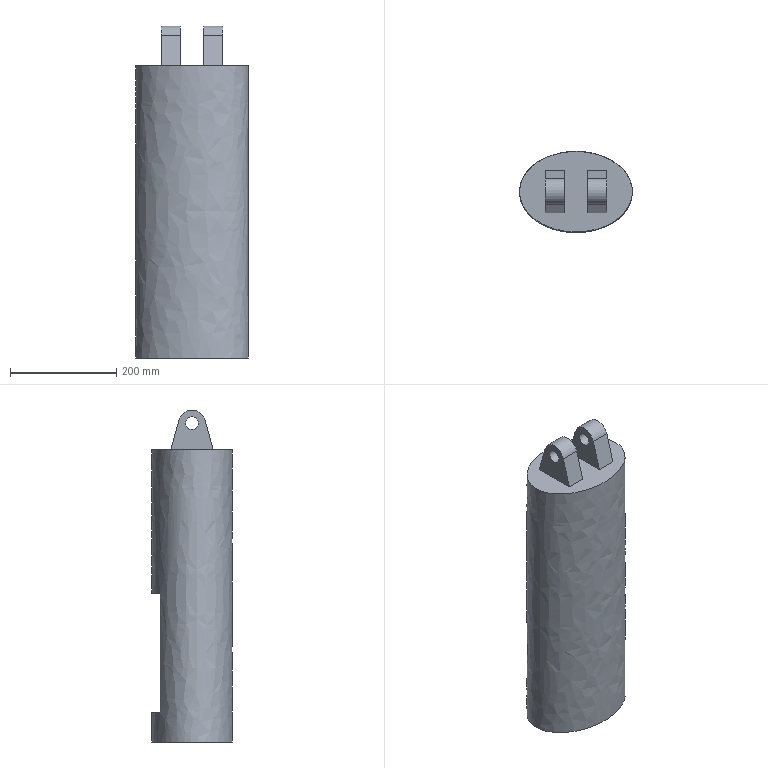Component | NX | UPPER_LINK_COLUMN | 1 solid | 28 faces | volume 13761102 mm3 | plane 18 | cylinder 9 | other 1 | commonest cylinder face diameters 30 x4 50 x2 24 x2 60 x1